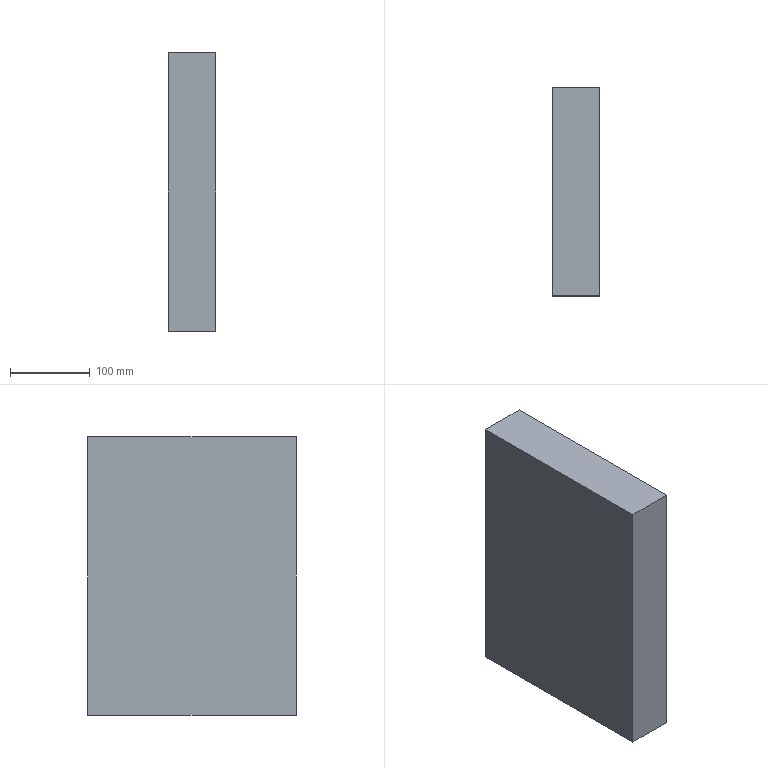Component | SolidWorks | Boss-1 | 1 solid | 6 faces | box 60 x 262 x 350 mm | volume 5502000 mm3 | plane 6
build123d program:
from build123d import *

# Parameters (mm, degrees)
SKETCH1_W           = 350
SKETCH1_H           = 262
BOSS_EXTRUDE1_DEPTH = 60


with BuildPart() as part:
    # Sketch1 → Boss-Extrude1 (new body)
    with BuildSketch(Plane(origin=(0, 0, 0), x_dir=(0, 0, -1), z_dir=(1, 0, 0))):
        Rectangle(SKETCH1_W, SKETCH1_H)
    extrude(amount=BOSS_EXTRUDE1_DEPTH)


solid = part.part

# Placed as in the assembly
solid = solid.moved(Location((-180.267, 15.31, -120), (0, 0, 0)))
STEP:
#1=COLOUR_RGB('',0.7922,0.8196,0.9333);
#2=FILL_AREA_STYLE_COLOUR('',#1);
#3=FILL_AREA_STYLE('',(#2));
#4=SURFACE_STYLE_FILL_AREA(#3);
#5=SURFACE_SIDE_STYLE('',(#4));
#6=SURFACE_STYLE_USAGE(.BOTH.,#5);
#7=PRESENTATION_STYLE_ASSIGNMENT((#6));
#8=CARTESIAN_POINT('',(-7.097,5.76,2.165));
#9=VERTEX_POINT('',#8);
#10=CARTESIAN_POINT('',(-7.097,-4.555,2.165));
#11=VERTEX_POINT('',#10);
#12=CARTESIAN_POINT('',(-7.097,5.76,2.165));
#13=DIRECTION('',(0.,-1.,-0.));
#14=VECTOR('',#13,39.37);
#15=LINE('',#12,#14);
#16=EDGE_CURVE('',#9,#11,#15,.T.);
#17=ORIENTED_EDGE('',*,*,#16,.T.);
#18=CARTESIAN_POINT('',(-4.735,-4.555,2.165));
#19=VERTEX_POINT('',#18);
#20=CARTESIAN_POINT('',(-4.735,-4.555,2.165));
#21=DIRECTION('',(-1.,0.,0.));
#22=VECTOR('',#21,39.37);
#23=LINE('',#20,#22);
#24=EDGE_CURVE('',#19,#11,#23,.T.);
#25=ORIENTED_EDGE('',*,*,#24,.F.);
#26=CARTESIAN_POINT('',(-4.735,5.76,2.165));
#27=VERTEX_POINT('',#26);
#28=CARTESIAN_POINT('',(-4.735,5.76,2.165));
#29=DIRECTION('',(0.,-1.,-0.));
#30=VECTOR('',#29,39.37);
#31=LINE('',#28,#30);
#32=EDGE_CURVE('',#27,#19,#31,.T.);
#33=ORIENTED_EDGE('',*,*,#32,.F.);
#34=CARTESIAN_POINT('',(-4.735,5.76,2.165));
#35=DIRECTION('',(-1.,0.,0.));
#36=VECTOR('',#35,39.37);
#37=LINE('',#34,#36);
#38=EDGE_CURVE('',#27,#9,#37,.T.);
#39=ORIENTED_EDGE('',*,*,#38,.T.);
#40=EDGE_LOOP('',(#17,#25,#33,#39));
#41=FACE_OUTER_BOUND('',#40,.T.);
#42=CARTESIAN_POINT('',(-4.735,5.76,2.165));
#43=DIRECTION('',(0.,0.,-1.));
#44=DIRECTION('',(0.,1.,0.));
#45=AXIS2_PLACEMENT_3D('',#42,#43,#44);
#46=PLANE('',#45);
#47=ADVANCED_FACE('',(#41),#46,.F.);
#48=CARTESIAN_POINT('',(-7.097,-4.555,-11.614));
#49=VERTEX_POINT('',#48);
#50=CARTESIAN_POINT('',(-7.097,-4.555,-11.614));
#51=DIRECTION('',(0.,0.,-1.));
#52=VECTOR('',#51,39.37);
#53=LINE('',#50,#52);
#54=EDGE_CURVE('',#11,#49,#53,.T.);
#55=ORIENTED_EDGE('',*,*,#54,.T.);
#56=CARTESIAN_POINT('',(-4.735,-4.555,-11.614));
#57=VERTEX_POINT('',#56);
#58=CARTESIAN_POINT('',(-4.735,-4.555,-11.614));
#59=DIRECTION('',(-1.,0.,0.));
#60=VECTOR('',#59,39.37);
#61=LINE('',#58,#60);
#62=EDGE_CURVE('',#57,#49,#61,.T.);
#63=ORIENTED_EDGE('',*,*,#62,.F.);
#64=CARTESIAN_POINT('',(-4.735,-4.555,-11.614));
#65=DIRECTION('',(0.,0.,-1.));
#66=VECTOR('',#65,39.37);
#67=LINE('',#64,#66);
#68=EDGE_CURVE('',#19,#57,#67,.T.);
#69=ORIENTED_EDGE('',*,*,#68,.F.);
#70=ORIENTED_EDGE('',*,*,#24,.T.);
#71=EDGE_LOOP('',(#55,#63,#69,#70));
#72=FACE_OUTER_BOUND('',#71,.T.);
#73=CARTESIAN_POINT('',(-4.735,-4.555,-11.614));
#74=DIRECTION('',(0.,1.,0.));
#75=DIRECTION('',(0.,-0.,1.));
#76=AXIS2_PLACEMENT_3D('',#73,#74,#75);
#77=PLANE('',#76);
#78=ADVANCED_FACE('',(#72),#77,.F.);
#79=CARTESIAN_POINT('',(-7.097,5.76,-11.614));
#80=VERTEX_POINT('',#79);
#81=CARTESIAN_POINT('',(-7.097,5.76,-11.614));
#82=DIRECTION('',(0.,1.,0.));
#83=VECTOR('',#82,39.37);
#84=LINE('',#81,#83);
#85=EDGE_CURVE('',#49,#80,#84,.T.);
#86=ORIENTED_EDGE('',*,*,#85,.T.);
#87=CARTESIAN_POINT('',(-4.735,5.76,-11.614));
#88=VERTEX_POINT('',#87);
#89=CARTESIAN_POINT('',(-4.735,5.76,-11.614));
#90=DIRECTION('',(-1.,0.,0.));
#91=VECTOR('',#90,39.37);
#92=LINE('',#89,#91);
#93=EDGE_CURVE('',#88,#80,#92,.T.);
#94=ORIENTED_EDGE('',*,*,#93,.F.);
#95=CARTESIAN_POINT('',(-4.735,5.76,-11.614));
#96=DIRECTION('',(0.,1.,0.));
#97=VECTOR('',#96,39.37);
#98=LINE('',#95,#97);
#99=EDGE_CURVE('',#57,#88,#98,.T.);
#100=ORIENTED_EDGE('',*,*,#99,.F.);
#101=ORIENTED_EDGE('',*,*,#62,.T.);
#102=EDGE_LOOP('',(#86,#94,#100,#101));
#103=FACE_OUTER_BOUND('',#102,.T.);
#104=CARTESIAN_POINT('',(-4.735,5.76,-11.614));
#105=DIRECTION('',(0.,-0.,1.));
#106=DIRECTION('',(0.,-1.,-0.));
#107=AXIS2_PLACEMENT_3D('',#104,#105,#106);
#108=PLANE('',#107);
#109=ADVANCED_FACE('',(#103),#108,.F.);
#110=CARTESIAN_POINT('',(-7.097,5.76,-11.614));
#111=DIRECTION('',(0.,-0.,1.));
#112=VECTOR('',#111,39.37);
#113=LINE('',#110,#112);
#114=EDGE_CURVE('',#80,#9,#113,.T.);
#115=ORIENTED_EDGE('',*,*,#114,.T.);
#116=ORIENTED_EDGE('',*,*,#38,.F.);
#117=CARTESIAN_POINT('',(-4.735,5.76,-11.614));
#118=DIRECTION('',(0.,-0.,1.));
#119=VECTOR('',#118,39.37);
#120=LINE('',#117,#119);
#121=EDGE_CURVE('',#88,#27,#120,.T.);
#122=ORIENTED_EDGE('',*,*,#121,.F.);
#123=ORIENTED_EDGE('',*,*,#93,.T.);
#124=EDGE_LOOP('',(#115,#116,#122,#123));
#125=FACE_OUTER_BOUND('',#124,.T.);
#126=CARTESIAN_POINT('',(-4.735,5.76,-11.614));
#127=DIRECTION('',(0.,-1.,-0.));
#128=DIRECTION('',(0.,0.,-1.));
#129=AXIS2_PLACEMENT_3D('',#126,#127,#128);
#130=PLANE('',#129);
#131=ADVANCED_FACE('',(#125),#130,.F.);
#132=ORIENTED_EDGE('',*,*,#32,.T.);
#133=ORIENTED_EDGE('',*,*,#68,.T.);
#134=ORIENTED_EDGE('',*,*,#99,.T.);
#135=ORIENTED_EDGE('',*,*,#121,.T.);
#136=EDGE_LOOP('',(#132,#133,#134,#135));
#137=FACE_OUTER_BOUND('',#136,.T.);
#138=CARTESIAN_POINT('',(-4.735,0.6028,-4.724));
#139=DIRECTION('',(-1.,0.,0.));
#140=DIRECTION('',(0.,0.,1.));
#141=AXIS2_PLACEMENT_3D('',#138,#139,#140);
#142=PLANE('',#141);
#143=ADVANCED_FACE('',(#137),#142,.F.);
#144=ORIENTED_EDGE('',*,*,#16,.F.);
#145=ORIENTED_EDGE('',*,*,#114,.F.);
#146=ORIENTED_EDGE('',*,*,#85,.F.);
#147=ORIENTED_EDGE('',*,*,#54,.F.);
#148=EDGE_LOOP('',(#144,#145,#146,#147));
#149=FACE_OUTER_BOUND('',#148,.T.);
#150=CARTESIAN_POINT('',(-7.097,0.6028,-4.724));
#151=DIRECTION('',(-1.,0.,0.));
#152=DIRECTION('',(0.,0.,1.));
#153=AXIS2_PLACEMENT_3D('',#150,#151,#152);
#154=PLANE('',#153);
#155=ADVANCED_FACE('',(#149),#154,.T.);
#156=CLOSED_SHELL('',(#47,#78,#109,#131,#143,#155));
#157=MANIFOLD_SOLID_BREP('',#156);
#158=STYLED_ITEM('',(#7),#157);
#159=(LENGTH_UNIT()NAMED_UNIT(*)SI_UNIT($,.METRE.));
#160=LENGTH_MEASURE_WITH_UNIT(LENGTH_MEASURE(0.0254),#159);
#161=DIMENSIONAL_EXPONENTS(1.,0.,0.,0.,0.,0.,0.);
#162=(CONVERSION_BASED_UNIT('',#160)LENGTH_UNIT()NAMED_UNIT(#161));
#163=UNCERTAINTY_MEASURE_WITH_UNIT(LENGTH_MEASURE(0.00001),#162,'','');
#164=(NAMED_UNIT(*)PLANE_ANGLE_UNIT()SI_UNIT($,.RADIAN.));
#165=(NAMED_UNIT(*)SI_UNIT($,.STERADIAN.)SOLID_ANGLE_UNIT());
#166=(GEOMETRIC_REPRESENTATION_CONTEXT(3)GLOBAL_UNCERTAINTY_ASSIGNED_CONTEXT((#163))GLOBAL_UNIT_ASSIGNED_CONTEXT((#162,#164,#165))REPRESENTATION_CONTEXT('',''));
#167=MECHANICAL_DESIGN_GEOMETRIC_PRESENTATION_REPRESENTATION('',(#158),#166);
#168=CARTESIAN_POINT('',(0.,0.,0.));
#169=DIRECTION('',(0.,0.,1.));
#170=DIRECTION('',(1.,0.,0.));
#171=AXIS2_PLACEMENT_3D('',#168,#169,#170);
#172=(LENGTH_UNIT()NAMED_UNIT(*)SI_UNIT($,.METRE.));
#173=LENGTH_MEASURE_WITH_UNIT(LENGTH_MEASURE(0.0254),#172);
#174=DIMENSIONAL_EXPONENTS(1.,0.,0.,0.,0.,0.,0.);
#175=(CONVERSION_BASED_UNIT('',#173)LENGTH_UNIT()NAMED_UNIT(#174));
#176=UNCERTAINTY_MEASURE_WITH_UNIT(LENGTH_MEASURE(0.00001),#175,'','');
#177=(NAMED_UNIT(*)PLANE_ANGLE_UNIT()SI_UNIT($,.RADIAN.));
#178=(NAMED_UNIT(*)SI_UNIT($,.STERADIAN.)SOLID_ANGLE_UNIT());
#179=(GEOMETRIC_REPRESENTATION_CONTEXT(3)GLOBAL_UNCERTAINTY_ASSIGNED_CONTEXT((#176))GLOBAL_UNIT_ASSIGNED_CONTEXT((#175,#177,#178))REPRESENTATION_CONTEXT('',''));
#180=ADVANCED_BREP_SHAPE_REPRESENTATION('',(#157,#171),#179);
#181=PRESENTATION_LAYER_ASSIGNMENT('','',(#158));